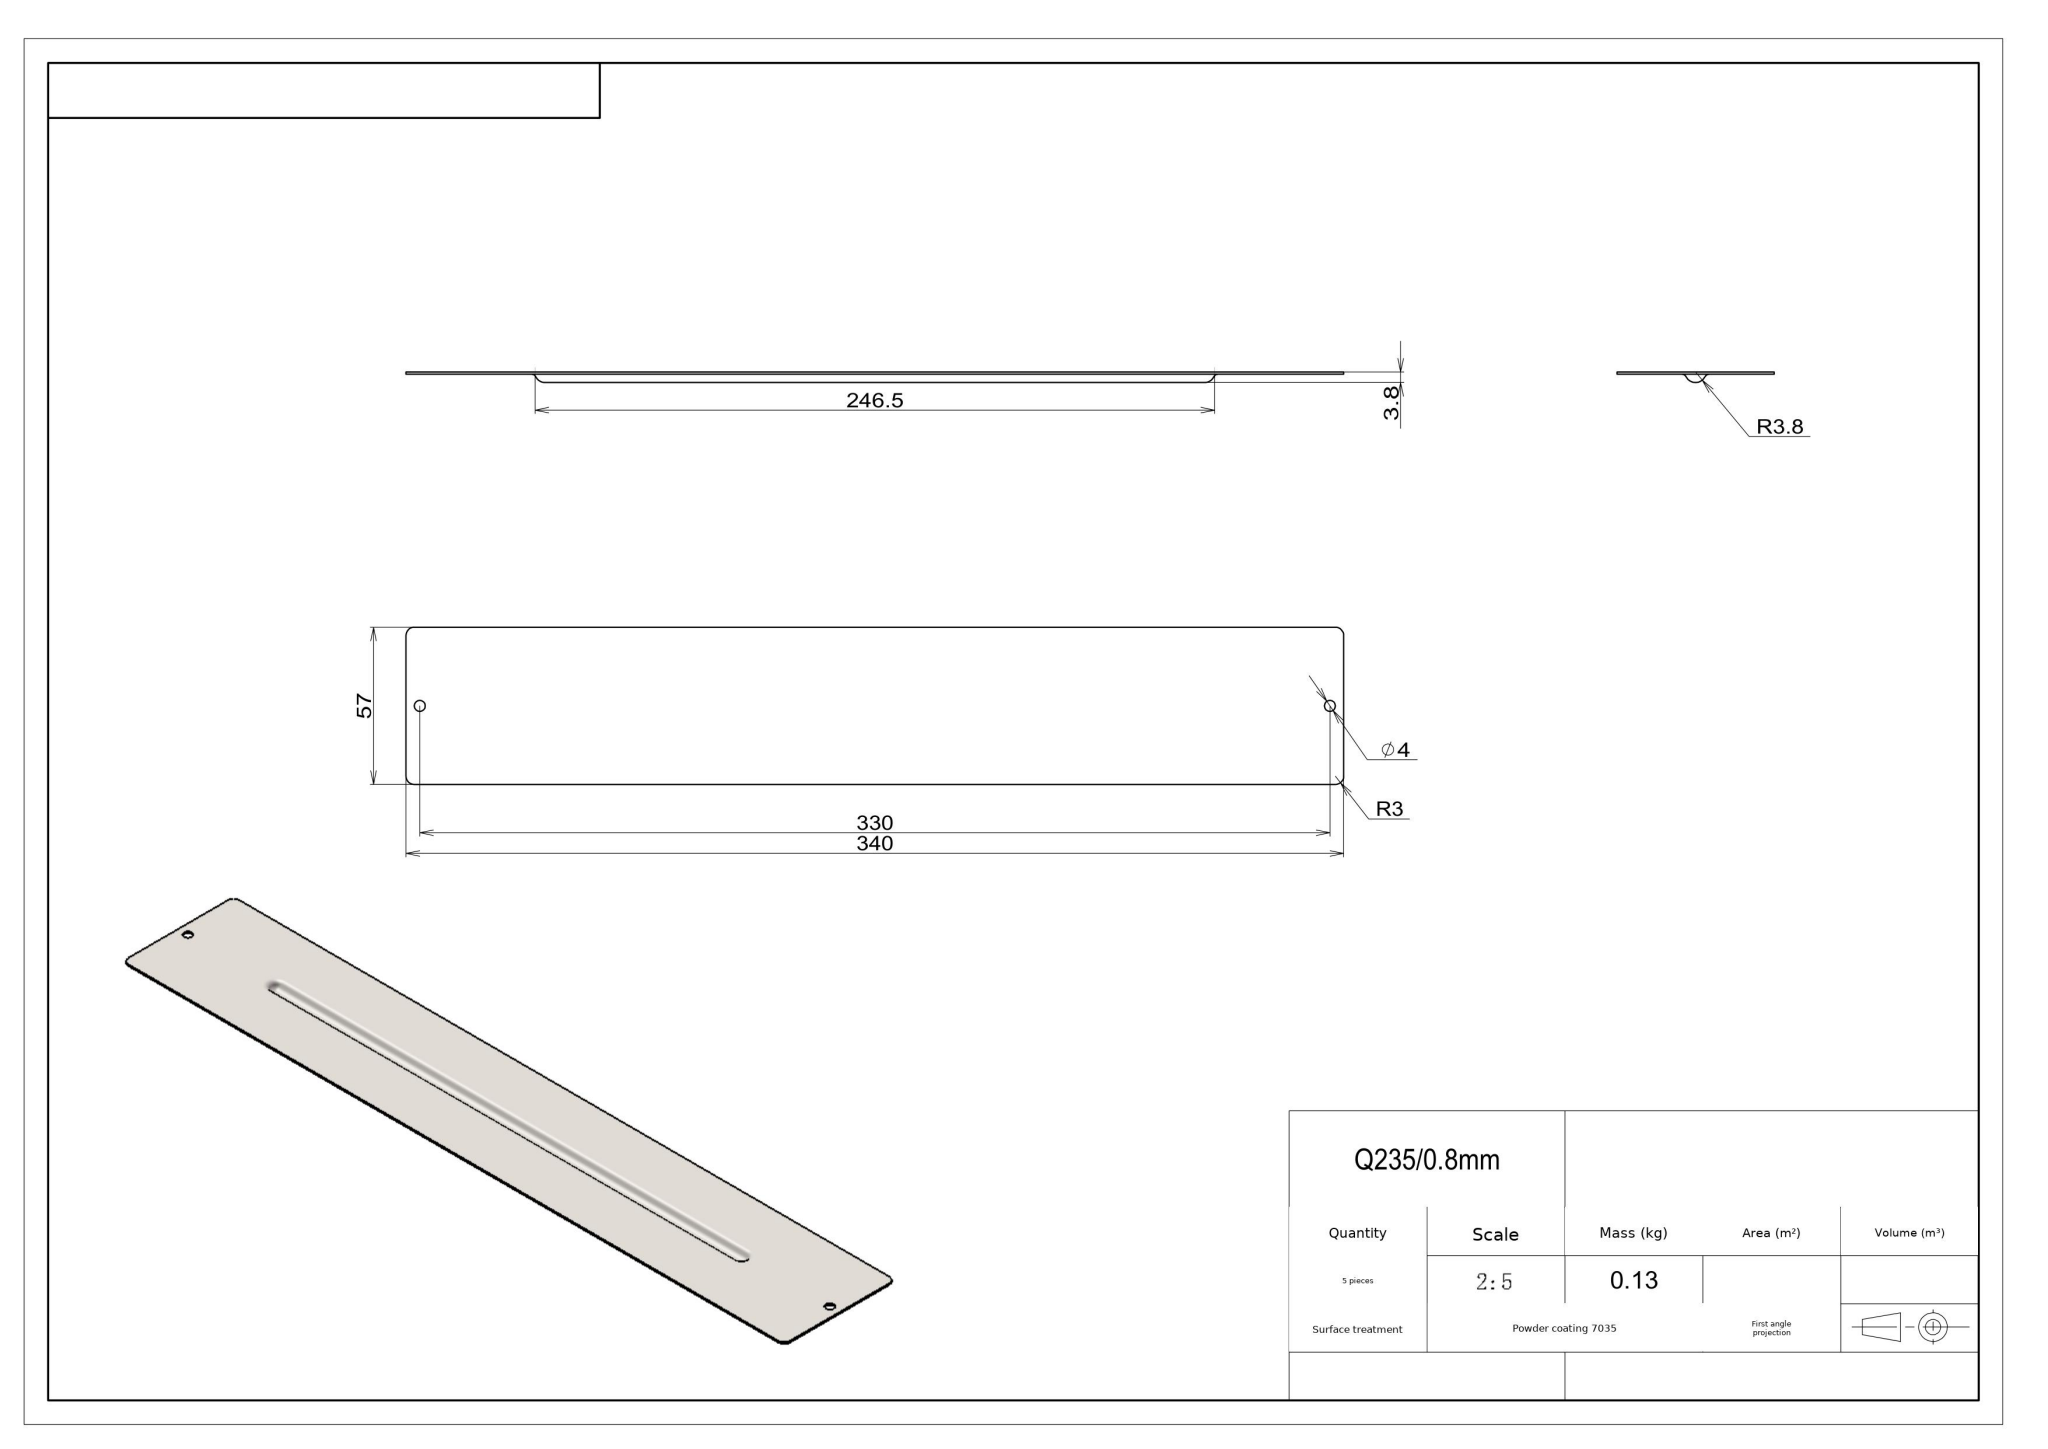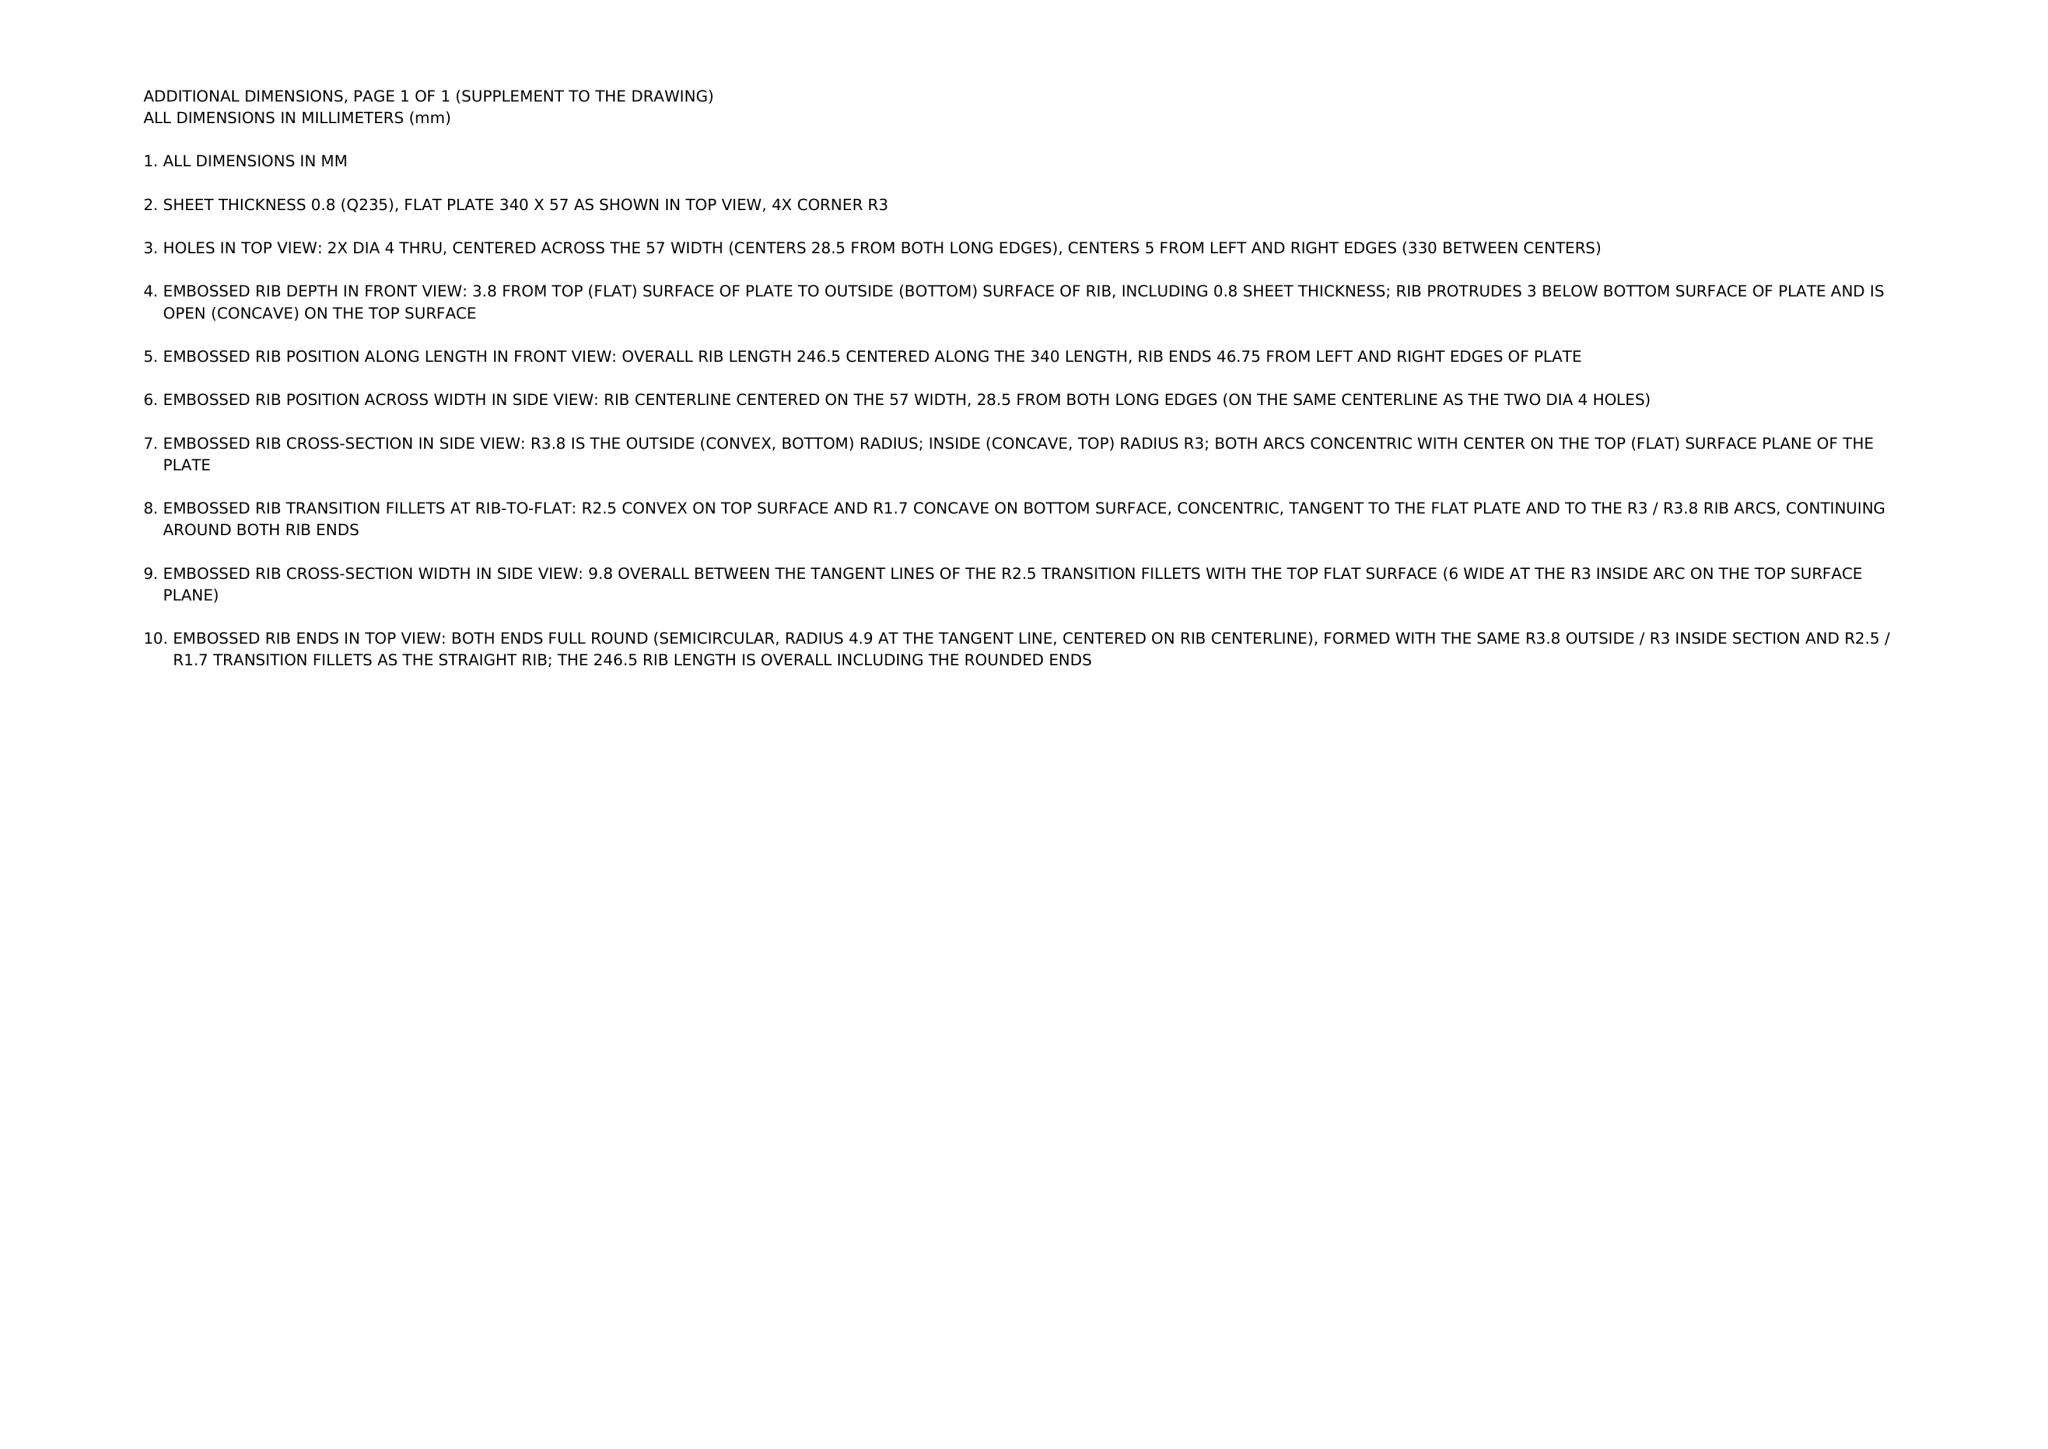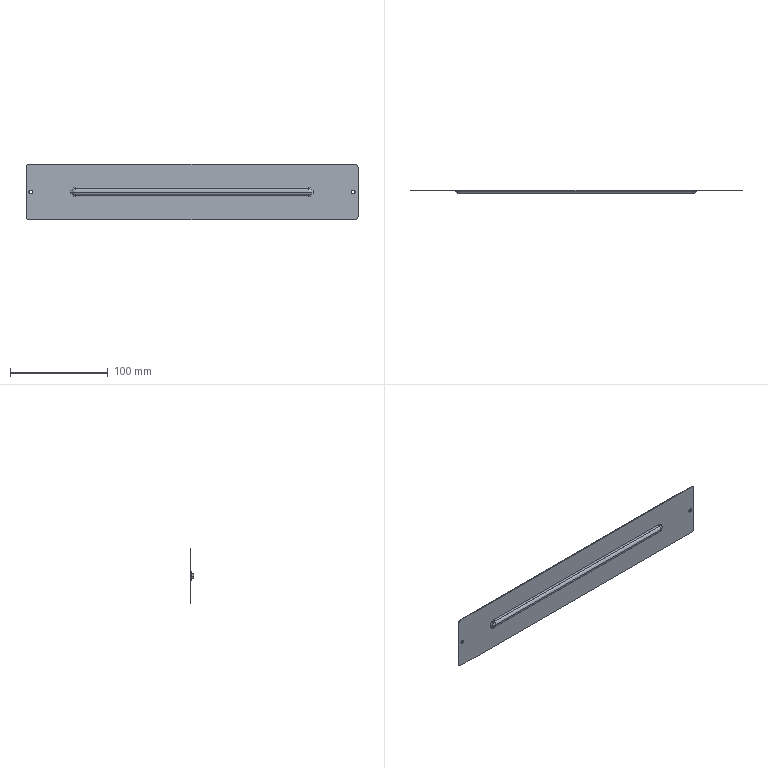Part | NX | mm | 1 solid | 36 faces | box 340 x 3.8 x 57 mm | volume 15932 mm3 | cylinder 16 | sphere 8 | torus 6 | plane 6 | commonest cylinder face diameters 6 x6 4 x4 7.6 x2 5 x2 3.4 x2